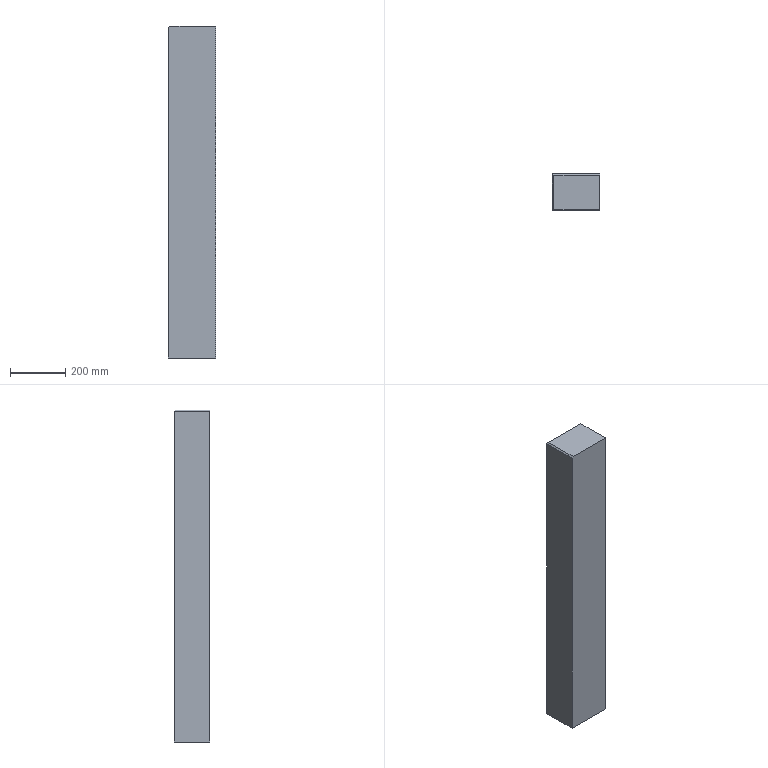Component | SolidWorks | Workpiece-1 | 1 solid | 8 faces | box 170 x 130 x 1200 mm | volume 26516292 mm3 | plane 8 | material Aviation Aluminum-7075
build123d program:
from build123d import *

# Parameters (mm, degrees)
SKETCH1_W           = 170
SKETCH1_H           = 130
BOSS_EXTRUDE1_DEPTH = 1200
CHAMFER1_SIZE       = 5


with BuildPart() as part:
    # Sketch1 → Boss-Extrude1 (new body)
    with BuildSketch(Plane.XY):
        Rectangle(SKETCH1_W, SKETCH1_H)
    extrude(amount=BOSS_EXTRUDE1_DEPTH)

    # Chamfer1
    chamfer1_edges = [part.edges().sort_by_distance(p)[0] for p in [
        (0, 65, 1200),
        (-85, 0, 1200),
    ]]
    chamfer(chamfer1_edges, length=CHAMFER1_SIZE)


solid = part.part

# Placed as in the assembly
solid = solid.moved(Location((-90.813, 248.429, -270), (0, 0, 0)))
STEP:
#1=COLOUR_RGB('',0.7922,0.8196,0.9333);
#2=FILL_AREA_STYLE_COLOUR('',#1);
#3=FILL_AREA_STYLE('',(#2));
#4=SURFACE_STYLE_FILL_AREA(#3);
#5=SURFACE_SIDE_STYLE('',(#4));
#6=SURFACE_STYLE_USAGE(.BOTH.,#5);
#7=PRESENTATION_STYLE_ASSIGNMENT((#6));
#8=CARTESIAN_POINT('',(-6.922,7.222,36.417));
#9=VERTEX_POINT('',#8);
#10=CARTESIAN_POINT('',(-6.922,7.222,-10.63));
#11=VERTEX_POINT('',#10);
#12=CARTESIAN_POINT('',(-6.922,7.222,36.614));
#13=DIRECTION('',(0.,0.,-1.));
#14=VECTOR('',#13,39.37);
#15=LINE('',#12,#14);
#16=EDGE_CURVE('',#9,#11,#15,.T.);
#17=ORIENTED_EDGE('',*,*,#16,.F.);
#18=CARTESIAN_POINT('',(-6.922,12.34,36.417));
#19=VERTEX_POINT('',#18);
#20=CARTESIAN_POINT('',(-6.922,12.34,36.417));
#21=DIRECTION('',(0.,1.,0.));
#22=VECTOR('',#21,39.37);
#23=LINE('',#20,#22);
#24=EDGE_CURVE('',#9,#19,#23,.T.);
#25=ORIENTED_EDGE('',*,*,#24,.T.);
#26=CARTESIAN_POINT('',(-6.922,12.34,-10.63));
#27=VERTEX_POINT('',#26);
#28=CARTESIAN_POINT('',(-6.922,12.34,36.614));
#29=DIRECTION('',(0.,0.,-1.));
#30=VECTOR('',#29,39.37);
#31=LINE('',#28,#30);
#32=EDGE_CURVE('',#19,#27,#31,.T.);
#33=ORIENTED_EDGE('',*,*,#32,.T.);
#34=CARTESIAN_POINT('',(-6.922,7.222,-10.63));
#35=DIRECTION('',(-0.,-1.,0.));
#36=VECTOR('',#35,39.37);
#37=LINE('',#34,#36);
#38=EDGE_CURVE('',#27,#11,#37,.T.);
#39=ORIENTED_EDGE('',*,*,#38,.T.);
#40=EDGE_LOOP('',(#17,#25,#33,#39));
#41=FACE_OUTER_BOUND('',#40,.T.);
#42=CARTESIAN_POINT('',(-6.922,7.222,36.614));
#43=DIRECTION('',(1.,-0.,0.));
#44=DIRECTION('',(0.,1.,0.));
#45=AXIS2_PLACEMENT_3D('',#42,#43,#44);
#46=PLANE('',#45);
#47=ADVANCED_FACE('',(#41),#46,.F.);
#48=CARTESIAN_POINT('',(-6.725,7.222,36.614));
#49=VERTEX_POINT('',#48);
#50=CARTESIAN_POINT('',(-0.2288,7.222,36.614));
#51=VERTEX_POINT('',#50);
#52=CARTESIAN_POINT('',(-0.2288,7.222,36.614));
#53=DIRECTION('',(1.,0.,0.));
#54=VECTOR('',#53,39.37);
#55=LINE('',#52,#54);
#56=EDGE_CURVE('',#49,#51,#55,.T.);
#57=ORIENTED_EDGE('',*,*,#56,.F.);
#58=CARTESIAN_POINT('',(-6.725,7.222,36.614));
#59=DIRECTION('',(-0.7071,-0.,-0.7071));
#60=VECTOR('',#59,39.37);
#61=LINE('',#58,#60);
#62=EDGE_CURVE('',#49,#9,#61,.T.);
#63=ORIENTED_EDGE('',*,*,#62,.T.);
#64=ORIENTED_EDGE('',*,*,#16,.T.);
#65=CARTESIAN_POINT('',(-0.2288,7.222,-10.63));
#66=VERTEX_POINT('',#65);
#67=CARTESIAN_POINT('',(-0.2288,7.222,-10.63));
#68=DIRECTION('',(1.,0.,0.));
#69=VECTOR('',#68,39.37);
#70=LINE('',#67,#69);
#71=EDGE_CURVE('',#11,#66,#70,.T.);
#72=ORIENTED_EDGE('',*,*,#71,.T.);
#73=CARTESIAN_POINT('',(-0.2288,7.222,36.614));
#74=DIRECTION('',(0.,0.,-1.));
#75=VECTOR('',#74,39.37);
#76=LINE('',#73,#75);
#77=EDGE_CURVE('',#51,#66,#76,.T.);
#78=ORIENTED_EDGE('',*,*,#77,.F.);
#79=EDGE_LOOP('',(#57,#63,#64,#72,#78));
#80=FACE_OUTER_BOUND('',#79,.T.);
#81=CARTESIAN_POINT('',(-0.2288,7.222,36.614));
#82=DIRECTION('',(-0.,1.,0.));
#83=DIRECTION('',(-1.,-0.,0.));
#84=AXIS2_PLACEMENT_3D('',#81,#82,#83);
#85=PLANE('',#84);
#86=ADVANCED_FACE('',(#80),#85,.F.);
#87=CARTESIAN_POINT('',(-0.2288,12.34,36.417));
#88=VERTEX_POINT('',#87);
#89=CARTESIAN_POINT('',(-0.2288,12.34,-10.63));
#90=VERTEX_POINT('',#89);
#91=CARTESIAN_POINT('',(-0.2288,12.34,36.614));
#92=DIRECTION('',(0.,0.,-1.));
#93=VECTOR('',#92,39.37);
#94=LINE('',#91,#93);
#95=EDGE_CURVE('',#88,#90,#94,.T.);
#96=ORIENTED_EDGE('',*,*,#95,.F.);
#97=CARTESIAN_POINT('',(-0.2288,12.143,36.614));
#98=VERTEX_POINT('',#97);
#99=CARTESIAN_POINT('',(-0.2288,12.143,36.614));
#100=DIRECTION('',(0.,-0.7071,0.7071));
#101=VECTOR('',#100,39.37);
#102=LINE('',#99,#101);
#103=EDGE_CURVE('',#88,#98,#102,.T.);
#104=ORIENTED_EDGE('',*,*,#103,.T.);
#105=CARTESIAN_POINT('',(-0.2288,7.222,36.614));
#106=DIRECTION('',(0.,1.,0.));
#107=VECTOR('',#106,39.37);
#108=LINE('',#105,#107);
#109=EDGE_CURVE('',#51,#98,#108,.T.);
#110=ORIENTED_EDGE('',*,*,#109,.F.);
#111=ORIENTED_EDGE('',*,*,#77,.T.);
#112=CARTESIAN_POINT('',(-0.2288,7.222,-10.63));
#113=DIRECTION('',(0.,1.,0.));
#114=VECTOR('',#113,39.37);
#115=LINE('',#112,#114);
#116=EDGE_CURVE('',#66,#90,#115,.T.);
#117=ORIENTED_EDGE('',*,*,#116,.T.);
#118=EDGE_LOOP('',(#96,#104,#110,#111,#117));
#119=FACE_OUTER_BOUND('',#118,.T.);
#120=CARTESIAN_POINT('',(-0.2288,7.222,36.614));
#121=DIRECTION('',(-1.,0.,0.));
#122=DIRECTION('',(0.,0.,1.));
#123=AXIS2_PLACEMENT_3D('',#120,#121,#122);
#124=PLANE('',#123);
#125=ADVANCED_FACE('',(#119),#124,.F.);
#126=ORIENTED_EDGE('',*,*,#32,.F.);
#127=CARTESIAN_POINT('',(-0.2288,12.34,36.417));
#128=DIRECTION('',(1.,0.,0.));
#129=VECTOR('',#128,39.37);
#130=LINE('',#127,#129);
#131=EDGE_CURVE('',#19,#88,#130,.T.);
#132=ORIENTED_EDGE('',*,*,#131,.T.);
#133=ORIENTED_EDGE('',*,*,#95,.T.);
#134=CARTESIAN_POINT('',(-0.2288,12.34,-10.63));
#135=DIRECTION('',(-1.,-0.,0.));
#136=VECTOR('',#135,39.37);
#137=LINE('',#134,#136);
#138=EDGE_CURVE('',#90,#27,#137,.T.);
#139=ORIENTED_EDGE('',*,*,#138,.T.);
#140=EDGE_LOOP('',(#126,#132,#133,#139));
#141=FACE_OUTER_BOUND('',#140,.T.);
#142=CARTESIAN_POINT('',(-0.2288,12.34,36.614));
#143=DIRECTION('',(0.,-1.,0.));
#144=DIRECTION('',(1.,0.,0.));
#145=AXIS2_PLACEMENT_3D('',#142,#143,#144);
#146=PLANE('',#145);
#147=ADVANCED_FACE('',(#141),#146,.F.);
#148=CARTESIAN_POINT('',(-6.725,12.143,36.614));
#149=VERTEX_POINT('',#148);
#150=CARTESIAN_POINT('',(-6.922,12.143,36.614));
#151=DIRECTION('',(-1.,-0.,0.));
#152=VECTOR('',#151,39.37);
#153=LINE('',#150,#152);
#154=EDGE_CURVE('',#98,#149,#153,.T.);
#155=ORIENTED_EDGE('',*,*,#154,.T.);
#156=CARTESIAN_POINT('',(-6.725,7.222,36.614));
#157=DIRECTION('',(-0.,-1.,0.));
#158=VECTOR('',#157,39.37);
#159=LINE('',#156,#158);
#160=EDGE_CURVE('',#149,#49,#159,.T.);
#161=ORIENTED_EDGE('',*,*,#160,.T.);
#162=ORIENTED_EDGE('',*,*,#56,.T.);
#163=ORIENTED_EDGE('',*,*,#109,.T.);
#164=EDGE_LOOP('',(#155,#161,#162,#163));
#165=FACE_OUTER_BOUND('',#164,.T.);
#166=CARTESIAN_POINT('',(-3.575,9.781,36.614));
#167=DIRECTION('',(0.,0.,1.));
#168=DIRECTION('',(1.,0.,0.));
#169=AXIS2_PLACEMENT_3D('',#166,#167,#168);
#170=PLANE('',#169);
#171=ADVANCED_FACE('',(#165),#170,.T.);
#172=ORIENTED_EDGE('',*,*,#38,.F.);
#173=ORIENTED_EDGE('',*,*,#138,.F.);
#174=ORIENTED_EDGE('',*,*,#116,.F.);
#175=ORIENTED_EDGE('',*,*,#71,.F.);
#176=EDGE_LOOP('',(#172,#173,#174,#175));
#177=FACE_OUTER_BOUND('',#176,.T.);
#178=CARTESIAN_POINT('',(-3.575,9.781,-10.63));
#179=DIRECTION('',(0.,0.,1.));
#180=DIRECTION('',(1.,0.,0.));
#181=AXIS2_PLACEMENT_3D('',#178,#179,#180);
#182=PLANE('',#181);
#183=ADVANCED_FACE('',(#177),#182,.F.);
#184=ORIENTED_EDGE('',*,*,#103,.F.);
#185=ORIENTED_EDGE('',*,*,#131,.F.);
#186=CARTESIAN_POINT('',(-5.675,11.093,37.664));
#187=DIRECTION('',(-0.5774,0.5774,-0.5774));
#188=VECTOR('',#187,39.37);
#189=LINE('',#186,#188);
#190=EDGE_CURVE('',#149,#19,#189,.T.);
#191=ORIENTED_EDGE('',*,*,#190,.F.);
#192=ORIENTED_EDGE('',*,*,#154,.F.);
#193=EDGE_LOOP('',(#184,#185,#191,#192));
#194=FACE_OUTER_BOUND('',#193,.T.);
#195=CARTESIAN_POINT('',(-3.575,12.143,36.614));
#196=DIRECTION('',(-0.,0.7071,0.7071));
#197=DIRECTION('',(1.,0.,0.));
#198=AXIS2_PLACEMENT_3D('',#195,#196,#197);
#199=PLANE('',#198);
#200=ADVANCED_FACE('',(#194),#199,.T.);
#201=ORIENTED_EDGE('',*,*,#190,.T.);
#202=ORIENTED_EDGE('',*,*,#24,.F.);
#203=ORIENTED_EDGE('',*,*,#62,.F.);
#204=ORIENTED_EDGE('',*,*,#160,.F.);
#205=EDGE_LOOP('',(#201,#202,#203,#204));
#206=FACE_OUTER_BOUND('',#205,.T.);
#207=CARTESIAN_POINT('',(-6.725,9.781,36.614));
#208=DIRECTION('',(-0.7071,0.,0.7071));
#209=DIRECTION('',(0.,1.,0.));
#210=AXIS2_PLACEMENT_3D('',#207,#208,#209);
#211=PLANE('',#210);
#212=ADVANCED_FACE('',(#206),#211,.T.);
#213=CLOSED_SHELL('',(#47,#86,#125,#147,#171,#183,#200,#212));
#214=MANIFOLD_SOLID_BREP('',#213);
#215=STYLED_ITEM('',(#7),#214);
#216=PRESENTATION_LAYER_ASSIGNMENT('','',(#215));
#217=(LENGTH_UNIT()NAMED_UNIT(*)SI_UNIT($,.METRE.));
#218=LENGTH_MEASURE_WITH_UNIT(LENGTH_MEASURE(0.0254),#217);
#219=DIMENSIONAL_EXPONENTS(1.,0.,0.,0.,0.,0.,0.);
#220=(CONVERSION_BASED_UNIT('',#218)LENGTH_UNIT()NAMED_UNIT(#219));
#221=UNCERTAINTY_MEASURE_WITH_UNIT(LENGTH_MEASURE(0.00001),#220,'','');
#222=(NAMED_UNIT(*)PLANE_ANGLE_UNIT()SI_UNIT($,.RADIAN.));
#223=(NAMED_UNIT(*)SI_UNIT($,.STERADIAN.)SOLID_ANGLE_UNIT());
#224=(GEOMETRIC_REPRESENTATION_CONTEXT(3)GLOBAL_UNCERTAINTY_ASSIGNED_CONTEXT((#221))GLOBAL_UNIT_ASSIGNED_CONTEXT((#220,#222,#223))REPRESENTATION_CONTEXT('',''));
#225=MECHANICAL_DESIGN_GEOMETRIC_PRESENTATION_REPRESENTATION('',(#215),#224);
#226=CARTESIAN_POINT('',(0.,0.,0.));
#227=DIRECTION('',(0.,0.,1.));
#228=DIRECTION('',(1.,0.,0.));
#229=AXIS2_PLACEMENT_3D('',#226,#227,#228);
#230=(LENGTH_UNIT()NAMED_UNIT(*)SI_UNIT($,.METRE.));
#231=LENGTH_MEASURE_WITH_UNIT(LENGTH_MEASURE(0.0254),#230);
#232=DIMENSIONAL_EXPONENTS(1.,0.,0.,0.,0.,0.,0.);
#233=(CONVERSION_BASED_UNIT('',#231)LENGTH_UNIT()NAMED_UNIT(#232));
#234=UNCERTAINTY_MEASURE_WITH_UNIT(LENGTH_MEASURE(0.00001),#233,'','');
#235=(NAMED_UNIT(*)PLANE_ANGLE_UNIT()SI_UNIT($,.RADIAN.));
#236=(NAMED_UNIT(*)SI_UNIT($,.STERADIAN.)SOLID_ANGLE_UNIT());
#237=(GEOMETRIC_REPRESENTATION_CONTEXT(3)GLOBAL_UNCERTAINTY_ASSIGNED_CONTEXT((#234))GLOBAL_UNIT_ASSIGNED_CONTEXT((#233,#235,#236))REPRESENTATION_CONTEXT('',''));
#238=ADVANCED_BREP_SHAPE_REPRESENTATION('',(#214,#229),#237);